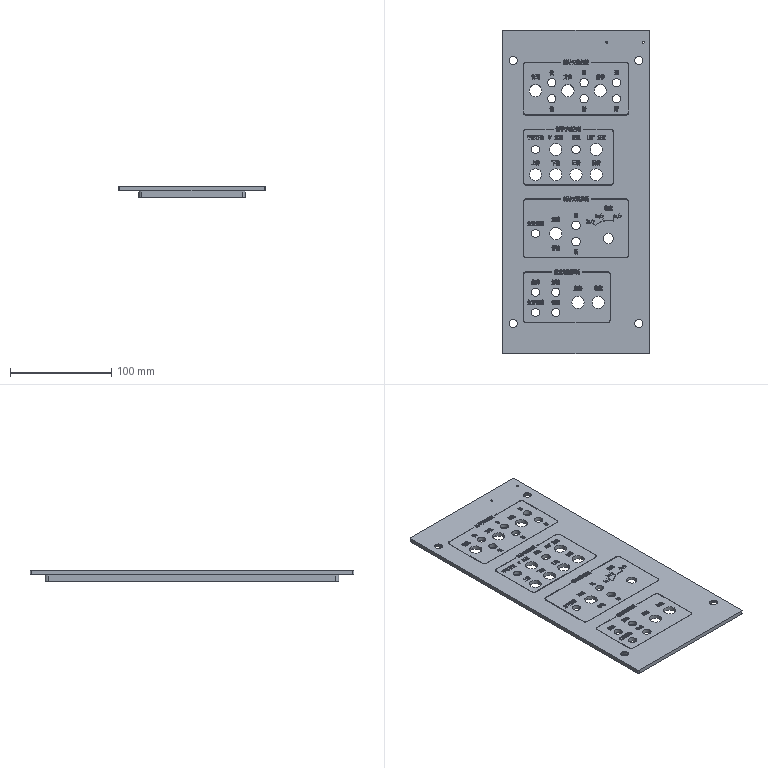CAM job | Mastercam | mm | 17 operations | part box 145 x 320 x 10
1. Contour (Ramp) | 9 - 10 平铣刀
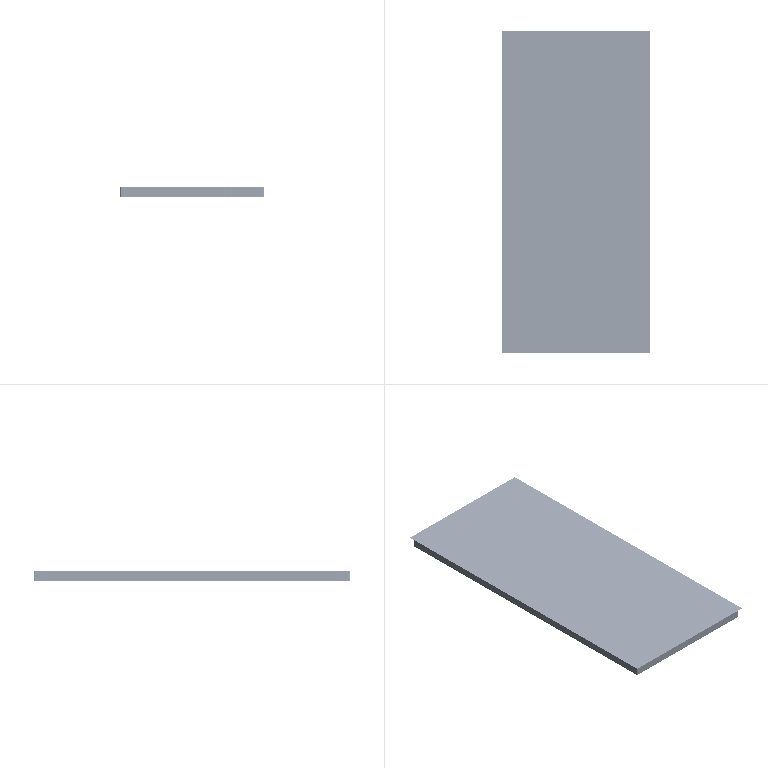2. 2D High Speed (2D Area Mill) | 9 - 10 平铣刀
3. 2D High Speed (2D Area Mill) | 9 - 10 平铣刀
4. Contour (2D) | 10 - 10 平铣刀
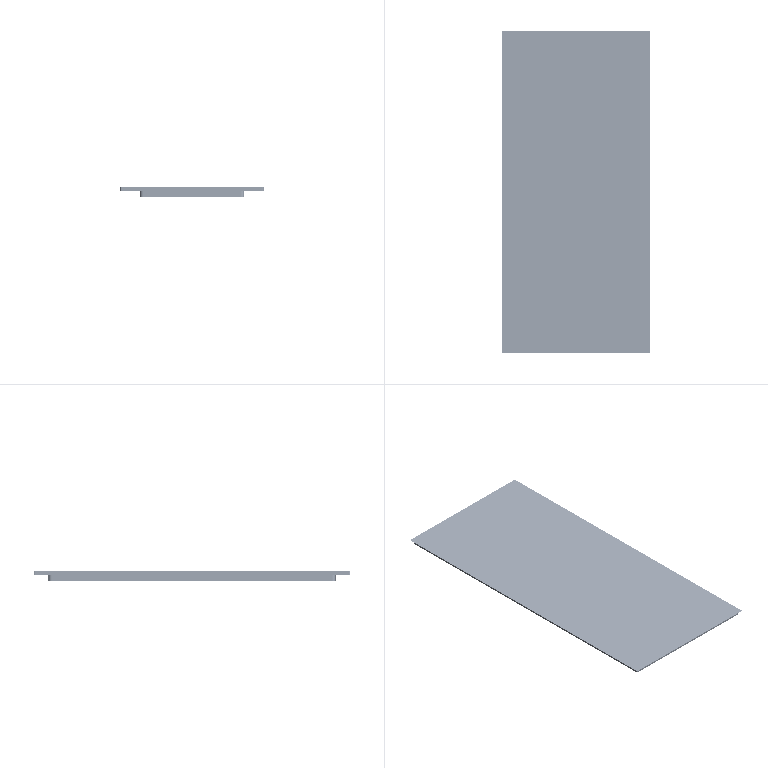5. 2D High Speed (2D Area Mill) | 10 - 10 平铣刀
6. Contour (Remachining) | 6 - 6 平铣刀
7. 2D High Speed (2D Area Mill) | 6 - 6 平铣刀
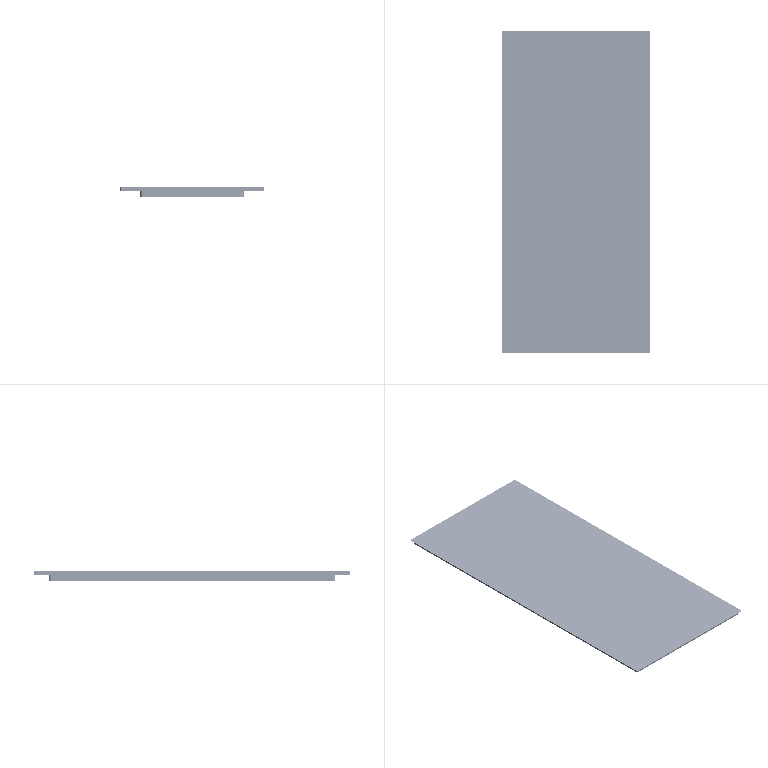8. Surface Finish Flowline | 4 - 4 平铣刀
9. Contour (Ramp) | 3 - 3 平铣刀
10. 2D High Speed (2D Area Mill) | 2 - 2 平铣刀
11. Contour (Ramp) | 2 - 2 平铣刀
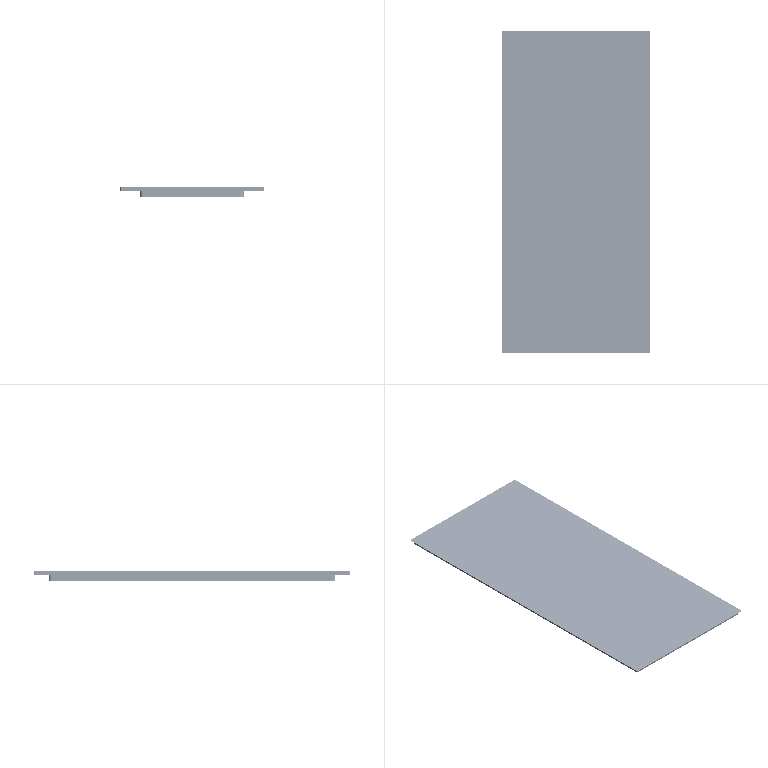12. Contour (2D) | 2 - 2 平铣刀
13. Contour (2D) | 2 - 2 平铣刀
14. Contour (Ramp) | 3 - 3 平铣刀
15. Drill/Counterbore | 5 - 4 倒角刀
16. Contour (2D chamfer) | 5 - 4 倒角刀
17. Contour (2D chamfer) | 5 - 4 倒角刀